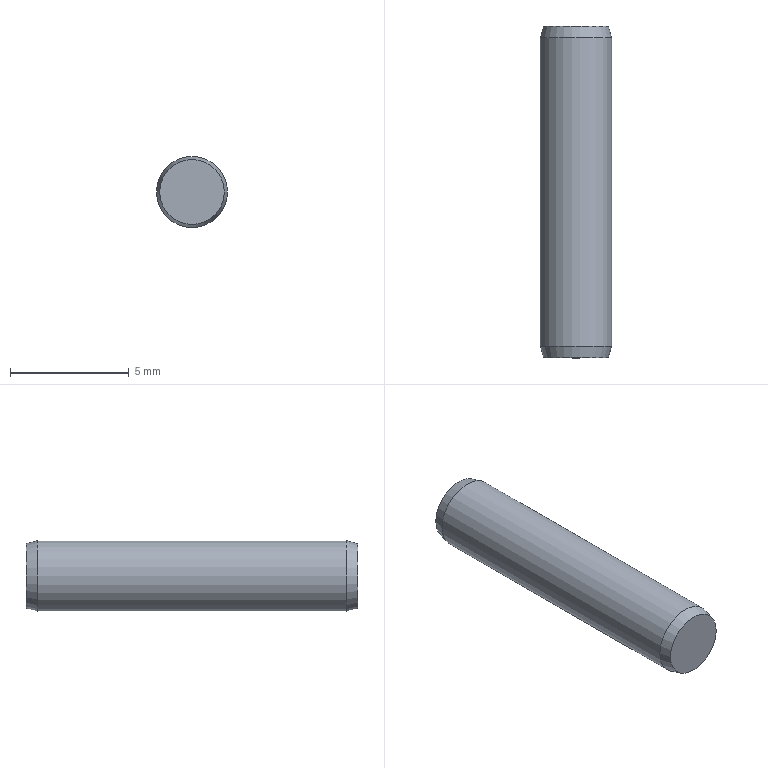Component | NX | PIN | 1 solid | 5 faces | box 3 x 14 x 3 mm | volume 98 mm3 | plane 2 | cone 2 | cylinder 1 | commonest cylinder face diameters 3 x1
STEP:
#1=CARTESIAN_POINT('',(0.,0.,0.));
#2=DIRECTION('',(0.,0.,1.));
#3=DIRECTION('',(1.,0.,0.));
#4=AXIS2_PLACEMENT_3D('',#1,#2,#3);
#5=CARTESIAN_POINT('',(18.866,-28.5,-25.811));
#6=VERTEX_POINT('',#5);
#7=CARTESIAN_POINT('',(17.5,-28.5,-25.811));
#8=DIRECTION('',(0.,1.,0.));
#9=DIRECTION('',(1.,0.,0.));
#10=AXIS2_PLACEMENT_3D('',#7,#8,#9);
#11=CIRCLE('',#10,1.366);
#12=CARTESIAN_POINT('',(17.5,-28.5,-25.811));
#13=DIRECTION('',(0.,1.,0.));
#14=DIRECTION('',(1.,0.,0.));
#15=AXIS2_PLACEMENT_3D('',#12,#13,#14);
#16=PLANE('',#15);
#17=CARTESIAN_POINT('',(0.,0.));
#18=DIRECTION('',(1.,0.));
#19=AXIS2_PLACEMENT_2D('',#17,#18);
#20=CIRCLE('',#19,1.366);
#21=(GEOMETRIC_REPRESENTATION_CONTEXT(2)PARAMETRIC_REPRESENTATION_CONTEXT()REPRESENTATION_CONTEXT('',''));
#22=DEFINITIONAL_REPRESENTATION('',(#20),#21);
#23=PCURVE('',#16,#22);
#24=CARTESIAN_POINT('',(17.5,-29.,-25.811));
#25=DIRECTION('',(0.,-1.,0.));
#26=DIRECTION('',(-1.,0.,0.));
#27=AXIS2_PLACEMENT_3D('',#24,#25,#26);
#28=CONICAL_SURFACE('',#27,1.5,0.2618);
#29=CARTESIAN_POINT('',(9.425,-0.5));
#30=DIRECTION('',(-1.,0.));
#31=VECTOR('',#30,1.);
#32=LINE('',#29,#31);
#33=(GEOMETRIC_REPRESENTATION_CONTEXT(2)PARAMETRIC_REPRESENTATION_CONTEXT()REPRESENTATION_CONTEXT('',''));
#34=DEFINITIONAL_REPRESENTATION('',(#32),#33);
#35=PCURVE('',#28,#34);
#36=SURFACE_CURVE('',#11,(#23,#35),.PCURVE_S1.);
#37=EDGE_CURVE('',#6,#6,#36,.T.);
#38=ORIENTED_EDGE('',*,*,#37,.T.);
#39=EDGE_LOOP('',(#38));
#40=FACE_BOUND('',#39,.T.);
#41=ADVANCED_FACE('',(#40),#16,.T.);
#42=CARTESIAN_POINT('',(16.134,-42.5,-25.811));
#43=VERTEX_POINT('',#42);
#44=CARTESIAN_POINT('',(17.5,-42.5,-25.811));
#45=DIRECTION('',(0.,-1.,0.));
#46=DIRECTION('',(-1.,0.,0.));
#47=AXIS2_PLACEMENT_3D('',#44,#45,#46);
#48=CIRCLE('',#47,1.366);
#49=CARTESIAN_POINT('',(17.5,-42.5,-25.811));
#50=DIRECTION('',(0.,-1.,0.));
#51=DIRECTION('',(-1.,0.,0.));
#52=AXIS2_PLACEMENT_3D('',#49,#50,#51);
#53=PLANE('',#52);
#54=CARTESIAN_POINT('',(0.,0.));
#55=DIRECTION('',(1.,0.));
#56=AXIS2_PLACEMENT_2D('',#54,#55);
#57=CIRCLE('',#56,1.366);
#58=(GEOMETRIC_REPRESENTATION_CONTEXT(2)PARAMETRIC_REPRESENTATION_CONTEXT()REPRESENTATION_CONTEXT('',''));
#59=DEFINITIONAL_REPRESENTATION('',(#57),#58);
#60=PCURVE('',#53,#59);
#61=CARTESIAN_POINT('',(17.5,-42.,-25.811));
#62=DIRECTION('',(0.,1.,0.));
#63=DIRECTION('',(1.,0.,0.));
#64=AXIS2_PLACEMENT_3D('',#61,#62,#63);
#65=CONICAL_SURFACE('',#64,1.5,0.2618);
#66=CARTESIAN_POINT('',(9.425,-0.5));
#67=DIRECTION('',(-1.,0.));
#68=VECTOR('',#67,1.);
#69=LINE('',#66,#68);
#70=(GEOMETRIC_REPRESENTATION_CONTEXT(2)PARAMETRIC_REPRESENTATION_CONTEXT()REPRESENTATION_CONTEXT('',''));
#71=DEFINITIONAL_REPRESENTATION('',(#69),#70);
#72=PCURVE('',#65,#71);
#73=SURFACE_CURVE('',#48,(#60,#72),.PCURVE_S1.);
#74=EDGE_CURVE('',#43,#43,#73,.T.);
#75=ORIENTED_EDGE('',*,*,#74,.T.);
#76=EDGE_LOOP('',(#75));
#77=FACE_BOUND('',#76,.T.);
#78=ADVANCED_FACE('',(#77),#53,.T.);
#79=CARTESIAN_POINT('',(16.,-42.,-25.811));
#80=VERTEX_POINT('',#79);
#81=CARTESIAN_POINT('',(19.,-42.,-25.811));
#82=VERTEX_POINT('',#81);
#83=CARTESIAN_POINT('',(17.5,-42.,-25.811));
#84=DIRECTION('',(0.,1.,0.));
#85=DIRECTION('',(-1.,0.,0.));
#86=AXIS2_PLACEMENT_3D('',#83,#84,#85);
#87=CIRCLE('',#86,1.5);
#88=CARTESIAN_POINT('',(17.5,-42.5,-25.811));
#89=DIRECTION('',(0.,1.,0.));
#90=DIRECTION('',(1.,0.,0.));
#91=AXIS2_PLACEMENT_3D('',#88,#89,#90);
#92=CYLINDRICAL_SURFACE('',#91,1.5);
#93=CARTESIAN_POINT('',(3.142,0.5));
#94=DIRECTION('',(1.,0.));
#95=VECTOR('',#94,1.);
#96=LINE('',#93,#95);
#97=(GEOMETRIC_REPRESENTATION_CONTEXT(2)PARAMETRIC_REPRESENTATION_CONTEXT()REPRESENTATION_CONTEXT('',''));
#98=DEFINITIONAL_REPRESENTATION('',(#96),#97);
#99=PCURVE('',#92,#98);
#100=CARTESIAN_POINT('',(3.142,0.));
#101=DIRECTION('',(1.,0.));
#102=VECTOR('',#101,1.);
#103=LINE('',#100,#102);
#104=(GEOMETRIC_REPRESENTATION_CONTEXT(2)PARAMETRIC_REPRESENTATION_CONTEXT()REPRESENTATION_CONTEXT('',''));
#105=DEFINITIONAL_REPRESENTATION('',(#103),#104);
#106=PCURVE('',#65,#105);
#107=SURFACE_CURVE('',#87,(#99,#106),.PCURVE_S1.);
#108=EDGE_CURVE('',#80,#82,#107,.T.);
#109=ORIENTED_EDGE('',*,*,#108,.T.);
#110=CARTESIAN_POINT('',(19.,-29.,-25.811));
#111=VERTEX_POINT('',#110);
#112=CARTESIAN_POINT('',(19.,-42.,-25.811));
#113=CARTESIAN_POINT('',(19.,-29.,-25.811));
#114=B_SPLINE_CURVE_WITH_KNOTS('',1,(#112,#113),.UNSPECIFIED.,.F.,.F.,(2,2),(0.5,13.5),.PIECEWISE_BEZIER_KNOTS.);
#115=CARTESIAN_POINT('',(6.283,0.));
#116=DIRECTION('',(0.,1.));
#117=VECTOR('',#116,1.);
#118=LINE('',#115,#117);
#119=(GEOMETRIC_REPRESENTATION_CONTEXT(2)PARAMETRIC_REPRESENTATION_CONTEXT()REPRESENTATION_CONTEXT('',''));
#120=DEFINITIONAL_REPRESENTATION('',(#118),#119);
#121=PCURVE('',#92,#120);
#122=CARTESIAN_POINT('',(0.,0.));
#123=DIRECTION('',(0.,1.));
#124=VECTOR('',#123,1.);
#125=LINE('',#122,#124);
#126=(GEOMETRIC_REPRESENTATION_CONTEXT(2)PARAMETRIC_REPRESENTATION_CONTEXT()REPRESENTATION_CONTEXT('',''));
#127=DEFINITIONAL_REPRESENTATION('',(#125),#126);
#128=PCURVE('',#92,#127);
#129=SEAM_CURVE('',#114,(#121,#128),.PCURVE_S1.);
#130=EDGE_CURVE('',#82,#111,#129,.T.);
#131=ORIENTED_EDGE('',*,*,#130,.T.);
#132=CARTESIAN_POINT('',(17.5,-29.,-25.811));
#133=DIRECTION('',(0.,-1.,0.));
#134=DIRECTION('',(1.,0.,0.));
#135=AXIS2_PLACEMENT_3D('',#132,#133,#134);
#136=CIRCLE('',#135,1.5);
#137=CARTESIAN_POINT('',(6.283,13.5));
#138=DIRECTION('',(-1.,0.));
#139=VECTOR('',#138,1.);
#140=LINE('',#137,#139);
#141=(GEOMETRIC_REPRESENTATION_CONTEXT(2)PARAMETRIC_REPRESENTATION_CONTEXT()REPRESENTATION_CONTEXT('',''));
#142=DEFINITIONAL_REPRESENTATION('',(#140),#141);
#143=PCURVE('',#92,#142);
#144=CARTESIAN_POINT('',(3.142,0.));
#145=DIRECTION('',(1.,0.));
#146=VECTOR('',#145,1.);
#147=LINE('',#144,#146);
#148=(GEOMETRIC_REPRESENTATION_CONTEXT(2)PARAMETRIC_REPRESENTATION_CONTEXT()REPRESENTATION_CONTEXT('',''));
#149=DEFINITIONAL_REPRESENTATION('',(#147),#148);
#150=PCURVE('',#28,#149);
#151=SURFACE_CURVE('',#136,(#143,#150),.PCURVE_S1.);
#152=EDGE_CURVE('',#111,#111,#151,.T.);
#153=ORIENTED_EDGE('',*,*,#152,.T.);
#154=ORIENTED_EDGE('',*,*,#130,.F.);
#155=CARTESIAN_POINT('',(17.5,-42.,-25.811));
#156=DIRECTION('',(0.,1.,0.));
#157=DIRECTION('',(-1.,0.,0.));
#158=AXIS2_PLACEMENT_3D('',#155,#156,#157);
#159=CIRCLE('',#158,1.5);
#160=CARTESIAN_POINT('',(-3.142,0.5));
#161=DIRECTION('',(1.,0.));
#162=VECTOR('',#161,1.);
#163=LINE('',#160,#162);
#164=(GEOMETRIC_REPRESENTATION_CONTEXT(2)PARAMETRIC_REPRESENTATION_CONTEXT()REPRESENTATION_CONTEXT('',''));
#165=DEFINITIONAL_REPRESENTATION('',(#163),#164);
#166=PCURVE('',#92,#165);
#167=CARTESIAN_POINT('',(3.142,0.));
#168=DIRECTION('',(1.,0.));
#169=VECTOR('',#168,1.);
#170=LINE('',#167,#169);
#171=(GEOMETRIC_REPRESENTATION_CONTEXT(2)PARAMETRIC_REPRESENTATION_CONTEXT()REPRESENTATION_CONTEXT('',''));
#172=DEFINITIONAL_REPRESENTATION('',(#170),#171);
#173=PCURVE('',#65,#172);
#174=SURFACE_CURVE('',#159,(#166,#173),.PCURVE_S1.);
#175=EDGE_CURVE('',#82,#80,#174,.T.);
#176=ORIENTED_EDGE('',*,*,#175,.T.);
#177=EDGE_LOOP('',(#109,#131,#153,#154,#176));
#178=FACE_BOUND('',#177,.T.);
#179=ADVANCED_FACE('',(#178),#92,.T.);
#180=ORIENTED_EDGE('',*,*,#74,.F.);
#181=CARTESIAN_POINT('',(16.134,-42.5,-25.811));
#182=CARTESIAN_POINT('',(16.,-42.,-25.811));
#183=B_SPLINE_CURVE_WITH_KNOTS('',1,(#181,#182),.UNSPECIFIED.,.F.,.F.,(2,2),(-0.5176,0.),.PIECEWISE_BEZIER_KNOTS.);
#184=CARTESIAN_POINT('',(9.425,0.));
#185=DIRECTION('',(0.,1.));
#186=VECTOR('',#185,1.);
#187=LINE('',#184,#186);
#188=(GEOMETRIC_REPRESENTATION_CONTEXT(2)PARAMETRIC_REPRESENTATION_CONTEXT()REPRESENTATION_CONTEXT('',''));
#189=DEFINITIONAL_REPRESENTATION('',(#187),#188);
#190=PCURVE('',#65,#189);
#191=CARTESIAN_POINT('',(3.142,0.));
#192=DIRECTION('',(0.,1.));
#193=VECTOR('',#192,1.);
#194=LINE('',#191,#193);
#195=(GEOMETRIC_REPRESENTATION_CONTEXT(2)PARAMETRIC_REPRESENTATION_CONTEXT()REPRESENTATION_CONTEXT('',''));
#196=DEFINITIONAL_REPRESENTATION('',(#194),#195);
#197=PCURVE('',#65,#196);
#198=SEAM_CURVE('',#183,(#190,#197),.PCURVE_S1.);
#199=EDGE_CURVE('',#43,#80,#198,.T.);
#200=ORIENTED_EDGE('',*,*,#199,.T.);
#201=ORIENTED_EDGE('',*,*,#175,.F.);
#202=ORIENTED_EDGE('',*,*,#108,.F.);
#203=ORIENTED_EDGE('',*,*,#199,.F.);
#204=EDGE_LOOP('',(#180,#200,#201,#202,#203));
#205=FACE_BOUND('',#204,.T.);
#206=ADVANCED_FACE('',(#205),#65,.T.);
#207=ORIENTED_EDGE('',*,*,#37,.F.);
#208=CARTESIAN_POINT('',(18.866,-28.5,-25.811));
#209=CARTESIAN_POINT('',(19.,-29.,-25.811));
#210=B_SPLINE_CURVE_WITH_KNOTS('',1,(#208,#209),.UNSPECIFIED.,.F.,.F.,(2,2),(-0.5176,0.),.PIECEWISE_BEZIER_KNOTS.);
#211=CARTESIAN_POINT('',(9.425,0.));
#212=DIRECTION('',(0.,1.));
#213=VECTOR('',#212,1.);
#214=LINE('',#211,#213);
#215=(GEOMETRIC_REPRESENTATION_CONTEXT(2)PARAMETRIC_REPRESENTATION_CONTEXT()REPRESENTATION_CONTEXT('',''));
#216=DEFINITIONAL_REPRESENTATION('',(#214),#215);
#217=PCURVE('',#28,#216);
#218=CARTESIAN_POINT('',(3.142,0.));
#219=DIRECTION('',(0.,1.));
#220=VECTOR('',#219,1.);
#221=LINE('',#218,#220);
#222=(GEOMETRIC_REPRESENTATION_CONTEXT(2)PARAMETRIC_REPRESENTATION_CONTEXT()REPRESENTATION_CONTEXT('',''));
#223=DEFINITIONAL_REPRESENTATION('',(#221),#222);
#224=PCURVE('',#28,#223);
#225=SEAM_CURVE('',#210,(#217,#224),.PCURVE_S1.);
#226=EDGE_CURVE('',#6,#111,#225,.T.);
#227=ORIENTED_EDGE('',*,*,#226,.T.);
#228=ORIENTED_EDGE('',*,*,#152,.F.);
#229=ORIENTED_EDGE('',*,*,#226,.F.);
#230=EDGE_LOOP('',(#207,#227,#228,#229));
#231=FACE_BOUND('',#230,.T.);
#232=ADVANCED_FACE('',(#231),#28,.T.);
#233=CLOSED_SHELL('',(#41,#78,#179,#206,#232));
#234=MANIFOLD_SOLID_BREP('',#233);
#235=(LENGTH_UNIT()NAMED_UNIT(*)SI_UNIT(.MILLI.,.METRE.));
#236=UNCERTAINTY_MEASURE_WITH_UNIT(LENGTH_MEASURE(0.00001),#235,'','');
#237=(NAMED_UNIT(*)PLANE_ANGLE_UNIT()SI_UNIT($,.RADIAN.));
#238=(NAMED_UNIT(*)SI_UNIT($,.STERADIAN.)SOLID_ANGLE_UNIT());
#239=(GEOMETRIC_REPRESENTATION_CONTEXT(3)GLOBAL_UNCERTAINTY_ASSIGNED_CONTEXT((#236))GLOBAL_UNIT_ASSIGNED_CONTEXT((#235,#237,#238))REPRESENTATION_CONTEXT('',''));
#240=ADVANCED_BREP_SHAPE_REPRESENTATION('',(#4,#234),#239);